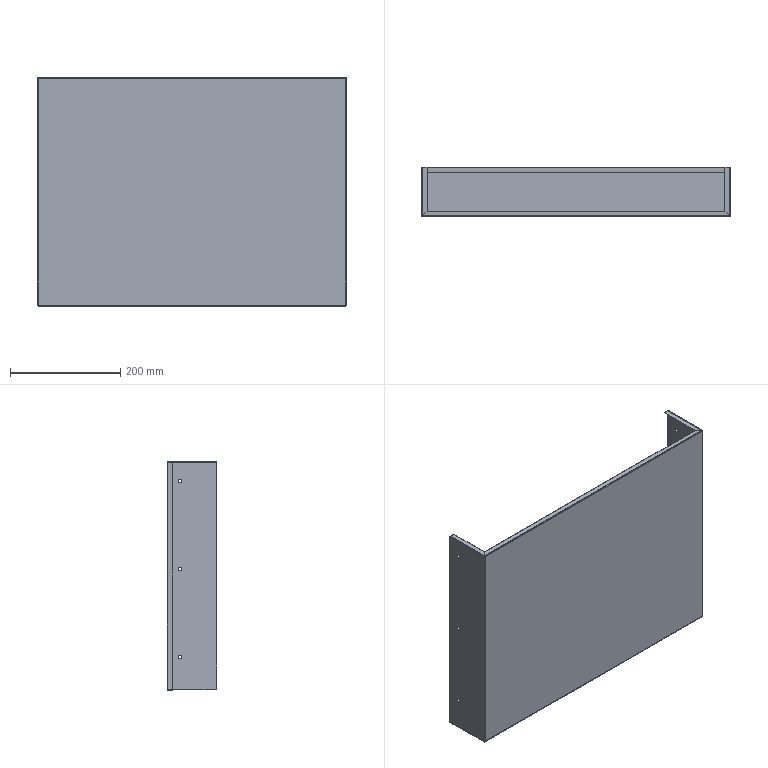Component | SolidWorks | PC-CAJ-P08-1_PC-CAJ-P17-2_PM-CAJ-P57-1 | 1 solid | 99 faces | volume 262694 mm3 | plane 62 | cylinder 33 | spline 4 | commonest cylinder face diameters 6 x12 1 x6 2.4 x6 1.6 x5 0.2 x4 | material Plain Carbon Steel